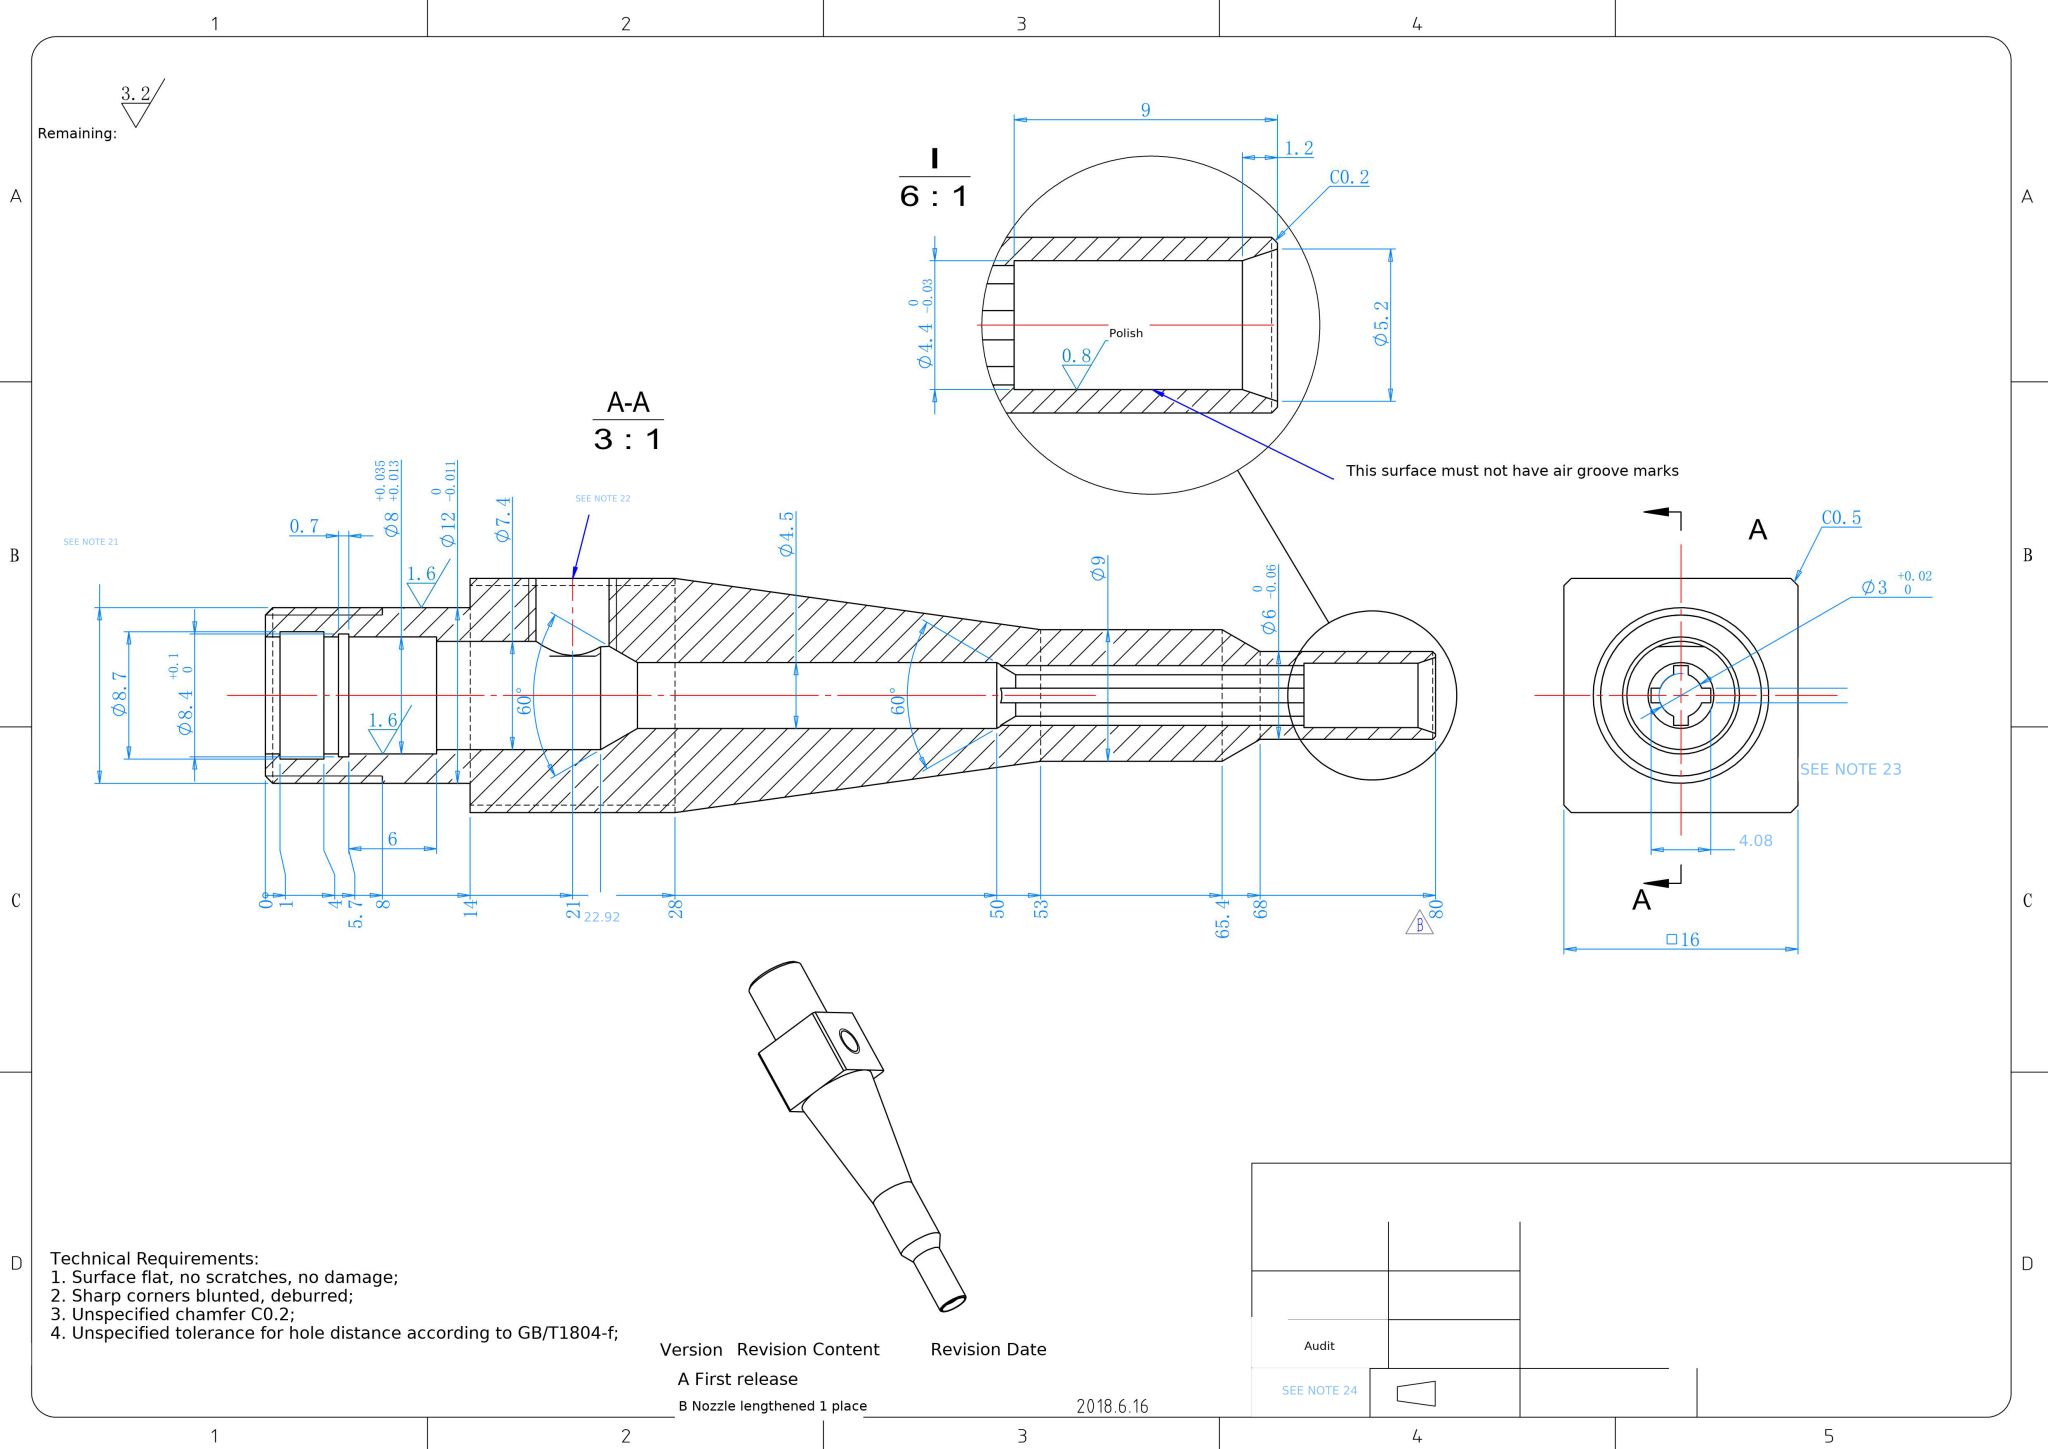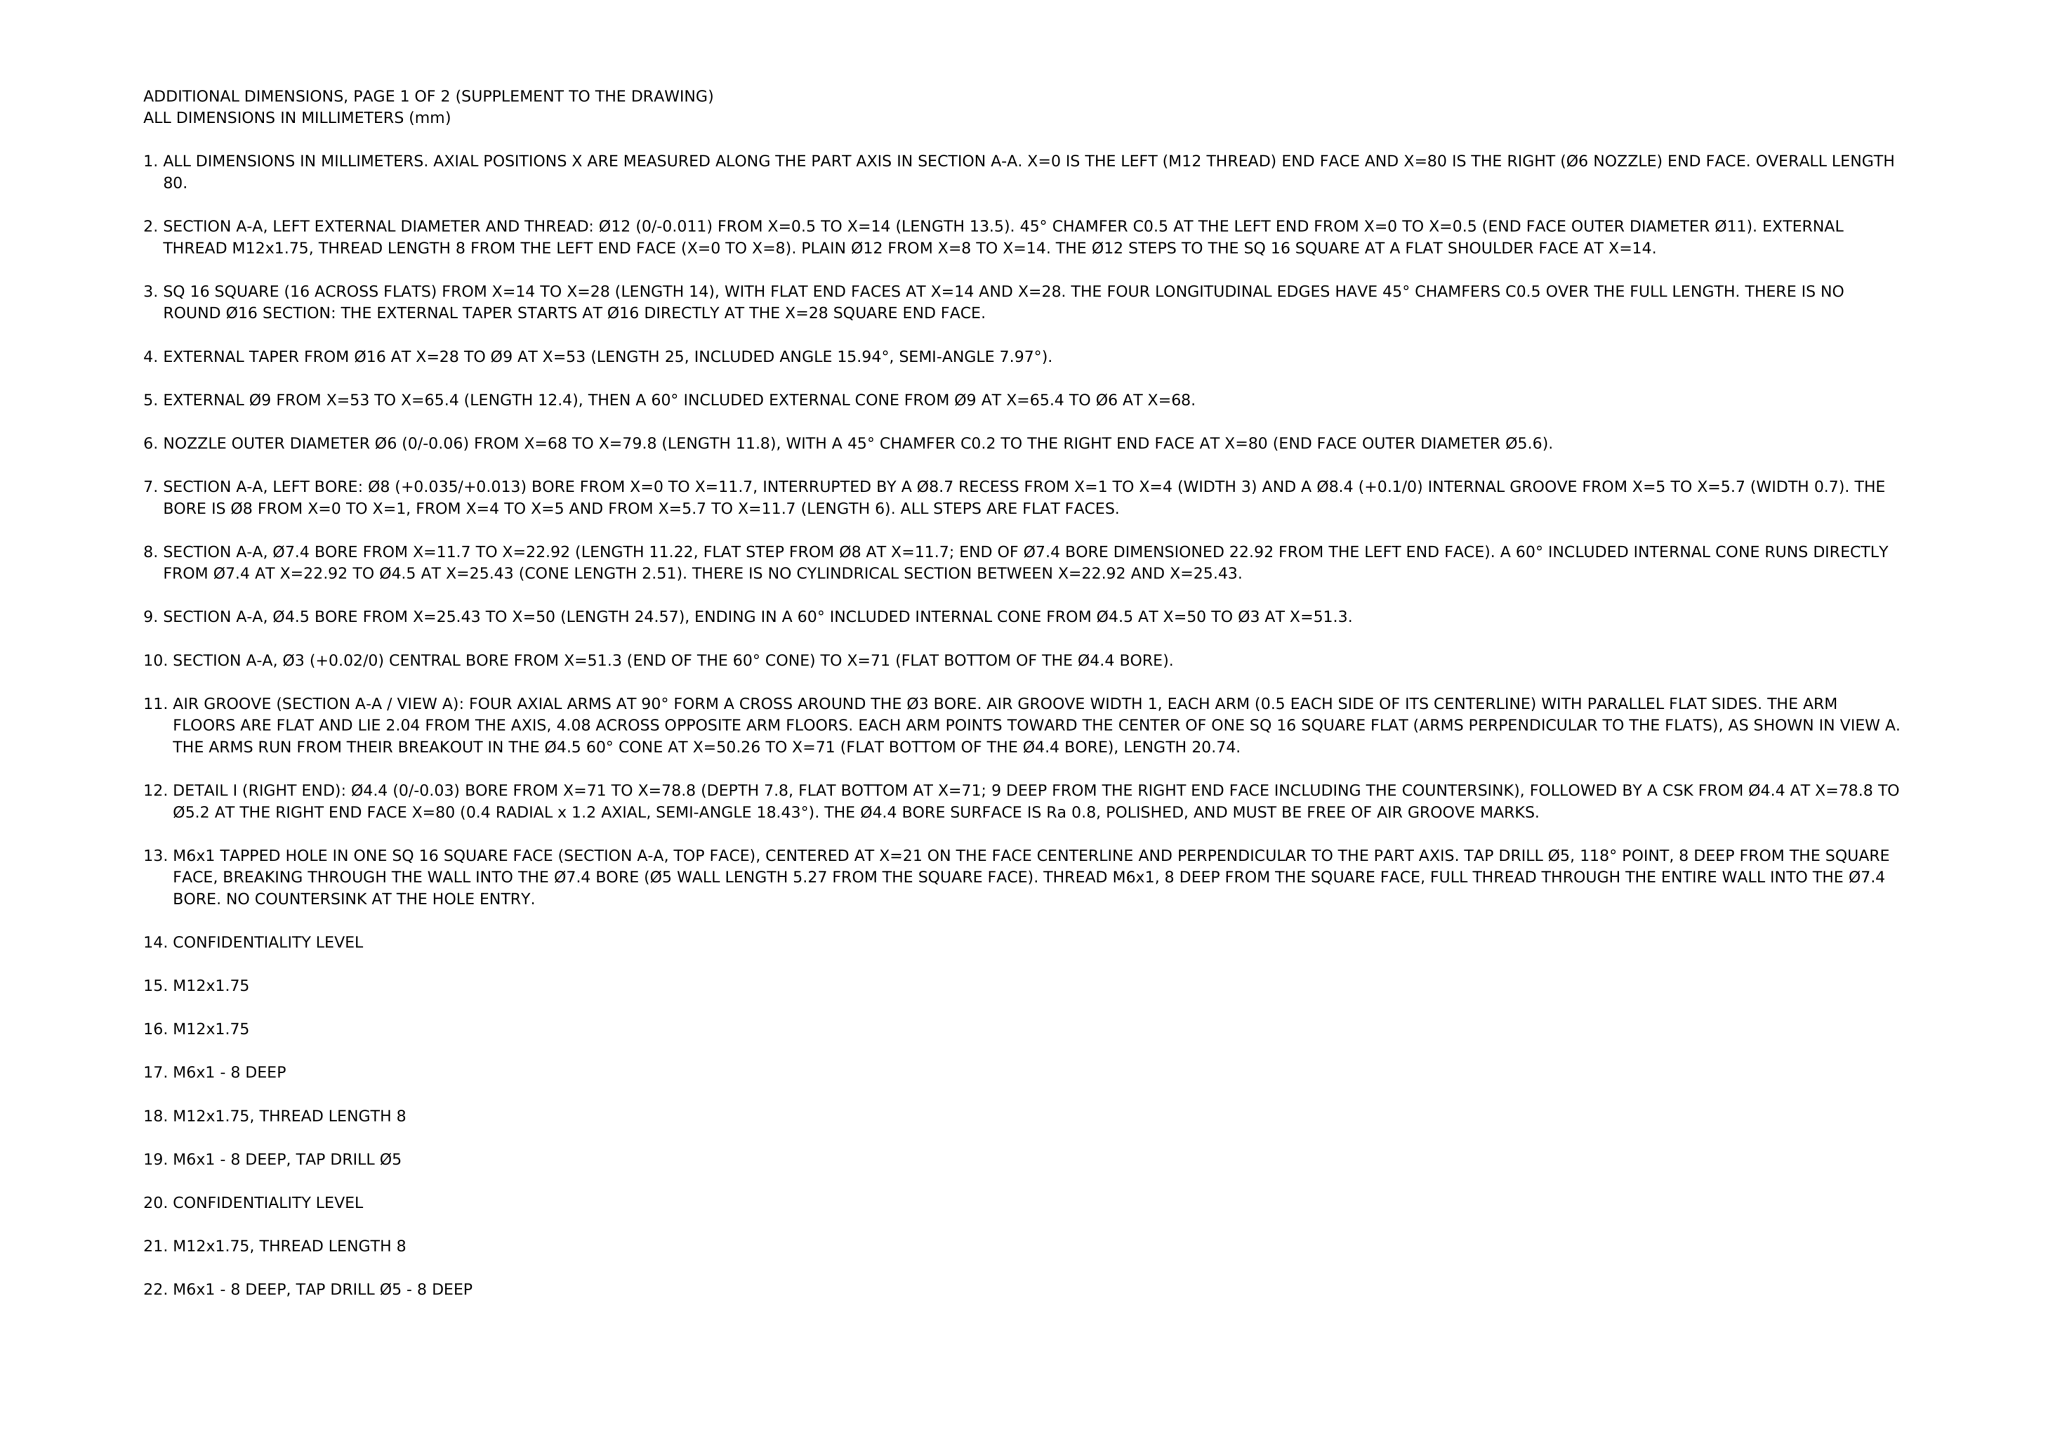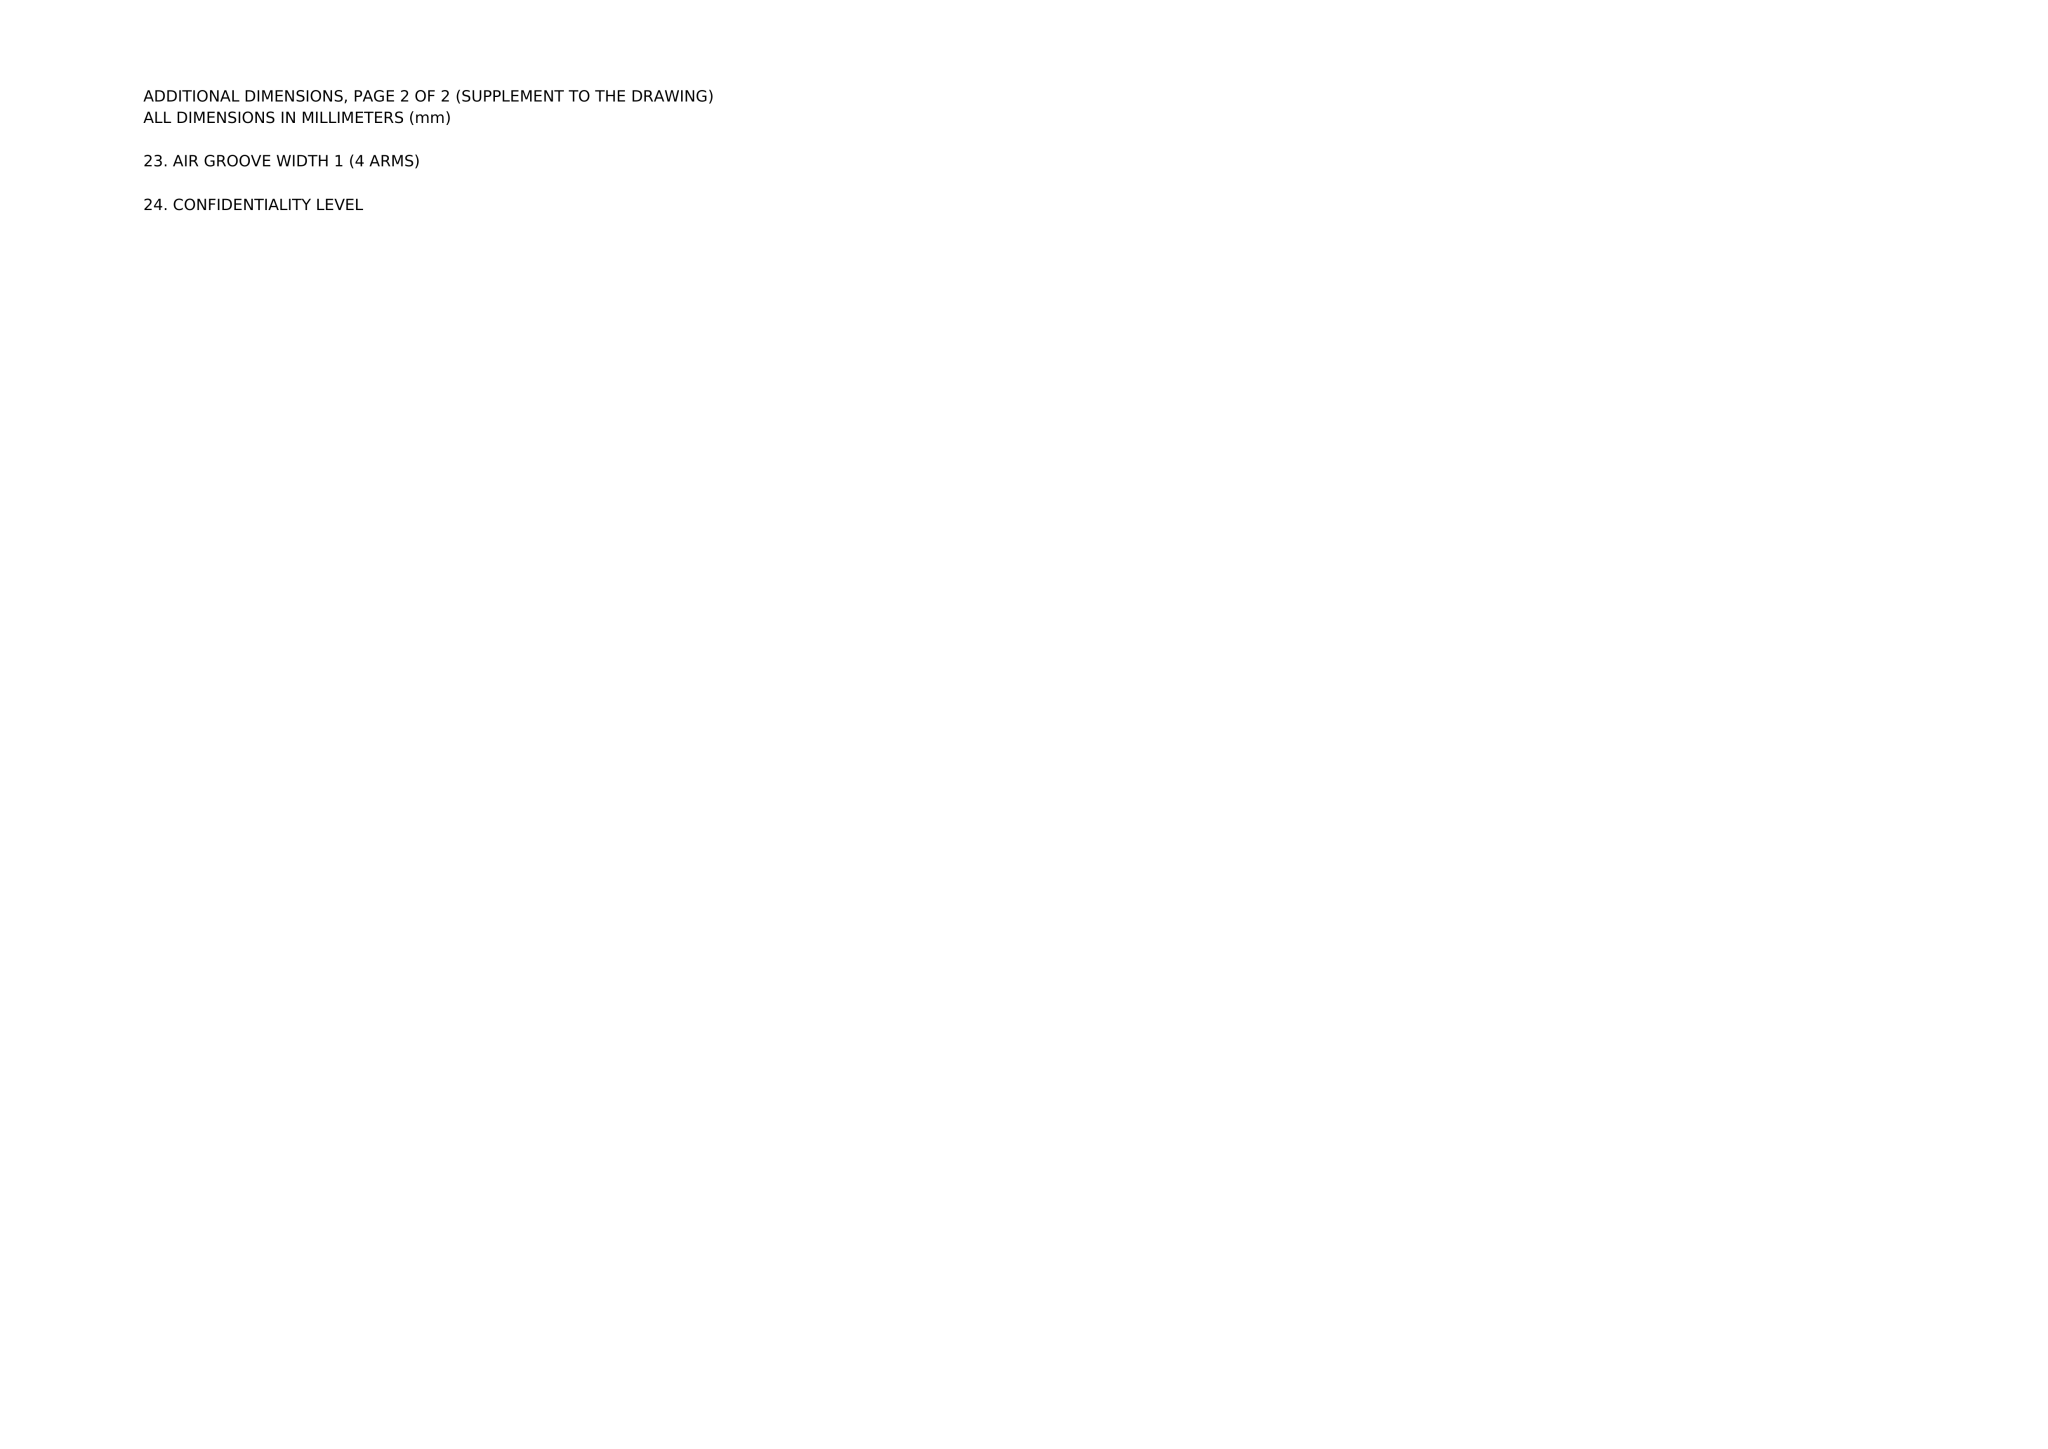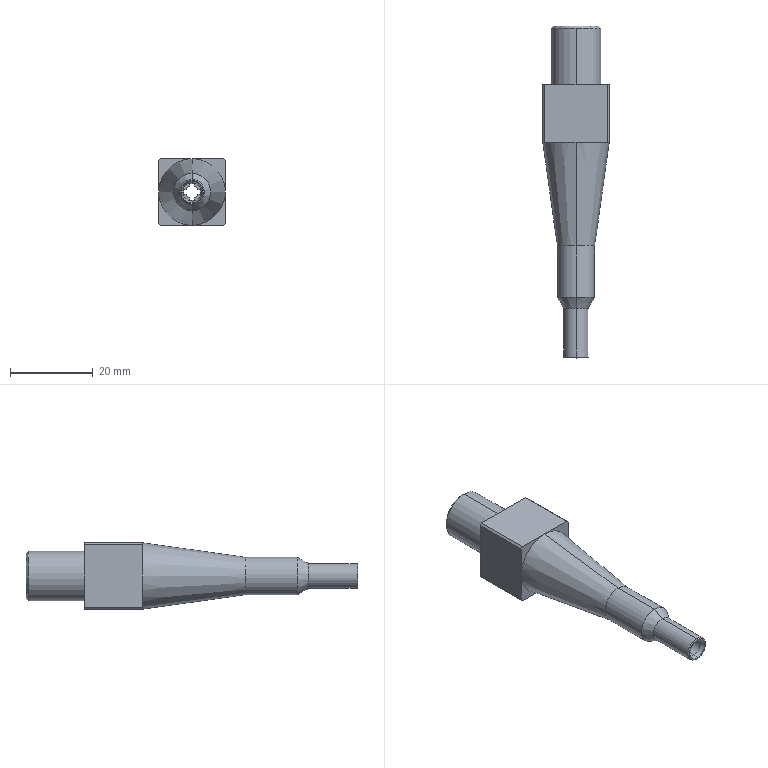Part | NX | mm | 1 solid | 75 faces | box 16 x 80 x 16 mm | volume 7555 mm3 | plane 33 | cylinder 28 | cone 14 | commonest cylinder face diameters 8 x6 3 x4 5 x2 9 x2 6 x2 4.4 x2 4.5 x2 7.4 x2